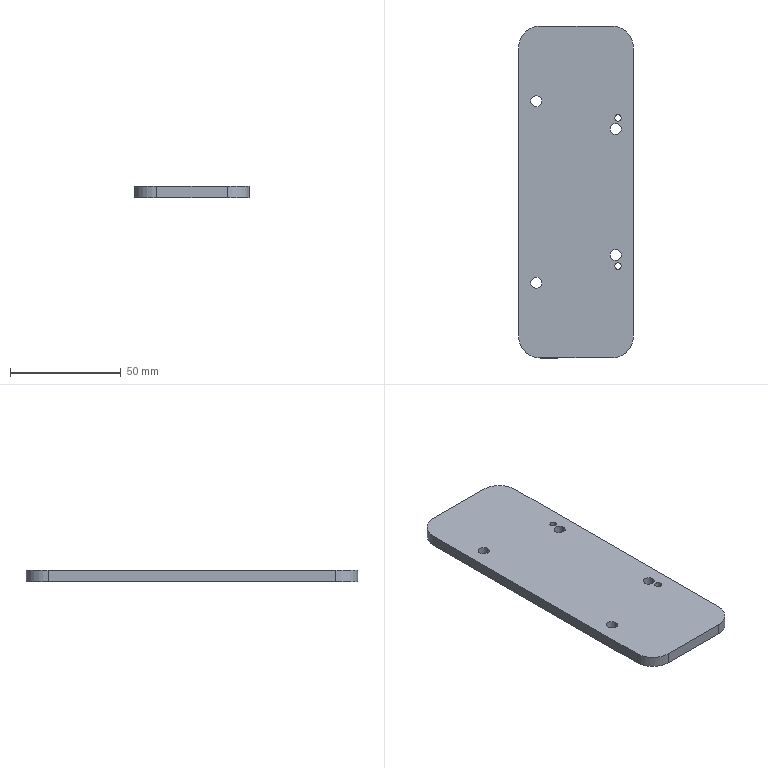Component | SolidWorks | MGL-PACK-03-00Fixture-1_MGL-PACK-03-02MovingPlate-1 | 1 solid | 22 faces | box 52 x 150 x 5 mm | volume 38107 mm3 | cylinder 16 | plane 6 | commonest cylinder face diameters 5 x8 3 x4 20 x4
build123d program:
from build123d import *

# Parameters (mm, degrees)
SKETCH1_W             = 52
SKETCH1_H             = 150
BOSS_EXTRUDE1_DEPTH   = 5
FILLET1_R             = 10
M5_TAPPED_HOLE1_D     = 5
M5_TAPPED_HOLE1_DEPTH = 14
M5_TAPPED_HOLE1_TIP   = 1.502
M3_TAPPED_HOLE1_D     = 3
M3_TAPPED_HOLE1_DEPTH = 8.5
M3_TAPPED_HOLE1_TIP   = 0.9013


with BuildPart() as part:
    # Sketch1 → Boss-Extrude1 (new body)
    with BuildSketch(Plane.XY):
        Rectangle(SKETCH1_W, SKETCH1_H)
    extrude(amount=BOSS_EXTRUDE1_DEPTH)

    # Fillet1
    fillet1_edges = [part.edges().sort_by_distance(p)[0] for p in [
        (-26, 75, 2.5),
        (26, 75, 2.5),
        (26, -75, 2.5),
        (-26, -75, 2.5),
    ]]
    fillet(fillet1_edges, radius=FILLET1_R)

    # M5 Tapped Hole1
    with Locations(Plane(origin=(0, 0, 0), x_dir=(-1, 0, 0), z_dir=(0, 0, -1))):
        with Locations((18, 41), (18, -41), (-18, -28.5), (-18, 28.5)):
            Hole(M5_TAPPED_HOLE1_D / 2, depth=M5_TAPPED_HOLE1_DEPTH)
            with Locations((0, 0, -(M5_TAPPED_HOLE1_DEPTH + M5_TAPPED_HOLE1_TIP / 2))):  # 118° drill point
                Cone(0, M5_TAPPED_HOLE1_D / 2, M5_TAPPED_HOLE1_TIP, mode=Mode.SUBTRACT)

    # M3 Tapped Hole1
    with Locations(Plane(origin=(0, 0, 0), x_dir=(-1, 0, 0), z_dir=(0, 0, -1))):
        with Locations((-19, 33.5), (-19, -33.5)):
            Hole(M3_TAPPED_HOLE1_D / 2, depth=M3_TAPPED_HOLE1_DEPTH)
            with Locations((0, 0, -(M3_TAPPED_HOLE1_DEPTH + M3_TAPPED_HOLE1_TIP / 2))):  # 118° drill point
                Cone(0, M3_TAPPED_HOLE1_D / 2, M3_TAPPED_HOLE1_TIP, mode=Mode.SUBTRACT)


solid = part.part

# Placed as in the assembly
solid = solid.moved(Location((248.5, 0, 13.7), (0, 0, 0)))
STEP:
#1=COLOUR_RGB('',0.7922,0.8196,0.9333);
#2=FILL_AREA_STYLE_COLOUR('',#1);
#3=FILL_AREA_STYLE('',(#2));
#4=SURFACE_STYLE_FILL_AREA(#3);
#5=SURFACE_SIDE_STYLE('',(#4));
#6=SURFACE_STYLE_USAGE(.BOTH.,#5);
#7=PRESENTATION_STYLE_ASSIGNMENT((#6));
#8=CARTESIAN_POINT('',(10.472,-1.319,0.5394));
#9=VERTEX_POINT('',#8);
#10=CARTESIAN_POINT('',(10.591,-1.319,0.5394));
#11=VERTEX_POINT('',#10);
#12=CARTESIAN_POINT('',(10.531,-1.319,0.5394));
#13=DIRECTION('',(-0.,-0.,-1.));
#14=DIRECTION('',(1.,0.,0.));
#15=AXIS2_PLACEMENT_3D('',#12,#13,#14);
#16=CIRCLE('',#15,0.05906);
#17=EDGE_CURVE('',#9,#11,#16,.T.);
#18=ORIENTED_EDGE('',*,*,#17,.T.);
#19=CARTESIAN_POINT('',(10.591,-1.319,0.7362));
#20=VERTEX_POINT('',#19);
#21=CARTESIAN_POINT('',(10.591,-1.319,0.7362));
#22=DIRECTION('',(0.,0.,1.));
#23=VECTOR('',#22,39.37);
#24=LINE('',#21,#23);
#25=EDGE_CURVE('',#11,#20,#24,.T.);
#26=ORIENTED_EDGE('',*,*,#25,.T.);
#27=CARTESIAN_POINT('',(10.472,-1.319,0.7362));
#28=VERTEX_POINT('',#27);
#29=CARTESIAN_POINT('',(10.531,-1.319,0.7362));
#30=DIRECTION('',(0.,0.,1.));
#31=DIRECTION('',(-1.,0.,0.));
#32=AXIS2_PLACEMENT_3D('',#29,#30,#31);
#33=CIRCLE('',#32,0.05906);
#34=EDGE_CURVE('',#20,#28,#33,.T.);
#35=ORIENTED_EDGE('',*,*,#34,.T.);
#36=CARTESIAN_POINT('',(10.472,-1.319,0.7362));
#37=DIRECTION('',(0.,0.,1.));
#38=VECTOR('',#37,39.37);
#39=LINE('',#36,#38);
#40=EDGE_CURVE('',#9,#28,#39,.T.);
#41=ORIENTED_EDGE('',*,*,#40,.F.);
#42=EDGE_LOOP('',(#18,#26,#35,#41));
#43=FACE_OUTER_BOUND('',#42,.T.);
#44=CARTESIAN_POINT('',(10.531,-1.319,0.7362));
#45=DIRECTION('',(0.,0.,1.));
#46=DIRECTION('',(-1.,0.,0.));
#47=AXIS2_PLACEMENT_3D('',#44,#45,#46);
#48=CYLINDRICAL_SURFACE('',#47,0.05906);
#49=ADVANCED_FACE('',(#43),#48,.F.);
#50=CARTESIAN_POINT('',(10.472,1.319,0.5394));
#51=VERTEX_POINT('',#50);
#52=CARTESIAN_POINT('',(10.591,1.319,0.5394));
#53=VERTEX_POINT('',#52);
#54=CARTESIAN_POINT('',(10.531,1.319,0.5394));
#55=DIRECTION('',(-0.,-0.,-1.));
#56=DIRECTION('',(1.,0.,0.));
#57=AXIS2_PLACEMENT_3D('',#54,#55,#56);
#58=CIRCLE('',#57,0.05906);
#59=EDGE_CURVE('',#51,#53,#58,.T.);
#60=ORIENTED_EDGE('',*,*,#59,.T.);
#61=CARTESIAN_POINT('',(10.591,1.319,0.7362));
#62=VERTEX_POINT('',#61);
#63=CARTESIAN_POINT('',(10.591,1.319,0.7362));
#64=DIRECTION('',(0.,0.,1.));
#65=VECTOR('',#64,39.37);
#66=LINE('',#63,#65);
#67=EDGE_CURVE('',#53,#62,#66,.T.);
#68=ORIENTED_EDGE('',*,*,#67,.T.);
#69=CARTESIAN_POINT('',(10.472,1.319,0.7362));
#70=VERTEX_POINT('',#69);
#71=CARTESIAN_POINT('',(10.531,1.319,0.7362));
#72=DIRECTION('',(0.,0.,1.));
#73=DIRECTION('',(-1.,0.,0.));
#74=AXIS2_PLACEMENT_3D('',#71,#72,#73);
#75=CIRCLE('',#74,0.05906);
#76=EDGE_CURVE('',#62,#70,#75,.T.);
#77=ORIENTED_EDGE('',*,*,#76,.T.);
#78=CARTESIAN_POINT('',(10.472,1.319,0.7362));
#79=DIRECTION('',(0.,0.,1.));
#80=VECTOR('',#79,39.37);
#81=LINE('',#78,#80);
#82=EDGE_CURVE('',#51,#70,#81,.T.);
#83=ORIENTED_EDGE('',*,*,#82,.F.);
#84=EDGE_LOOP('',(#60,#68,#77,#83));
#85=FACE_OUTER_BOUND('',#84,.T.);
#86=CARTESIAN_POINT('',(10.531,1.319,0.7362));
#87=DIRECTION('',(0.,0.,1.));
#88=DIRECTION('',(-1.,0.,0.));
#89=AXIS2_PLACEMENT_3D('',#86,#87,#88);
#90=CYLINDRICAL_SURFACE('',#89,0.05906);
#91=ADVANCED_FACE('',(#85),#90,.F.);
#92=CARTESIAN_POINT('',(8.976,-1.614,0.5394));
#93=VERTEX_POINT('',#92);
#94=CARTESIAN_POINT('',(9.173,-1.614,0.5394));
#95=VERTEX_POINT('',#94);
#96=CARTESIAN_POINT('',(9.075,-1.614,0.5394));
#97=DIRECTION('',(-0.,-0.,-1.));
#98=DIRECTION('',(1.,0.,0.));
#99=AXIS2_PLACEMENT_3D('',#96,#97,#98);
#100=CIRCLE('',#99,0.09843);
#101=EDGE_CURVE('',#93,#95,#100,.T.);
#102=ORIENTED_EDGE('',*,*,#101,.T.);
#103=CARTESIAN_POINT('',(9.173,-1.614,0.7362));
#104=VERTEX_POINT('',#103);
#105=CARTESIAN_POINT('',(9.173,-1.614,0.7362));
#106=DIRECTION('',(0.,0.,1.));
#107=VECTOR('',#106,39.37);
#108=LINE('',#105,#107);
#109=EDGE_CURVE('',#95,#104,#108,.T.);
#110=ORIENTED_EDGE('',*,*,#109,.T.);
#111=CARTESIAN_POINT('',(8.976,-1.614,0.7362));
#112=VERTEX_POINT('',#111);
#113=CARTESIAN_POINT('',(9.075,-1.614,0.7362));
#114=DIRECTION('',(0.,0.,1.));
#115=DIRECTION('',(-1.,0.,0.));
#116=AXIS2_PLACEMENT_3D('',#113,#114,#115);
#117=CIRCLE('',#116,0.09843);
#118=EDGE_CURVE('',#104,#112,#117,.T.);
#119=ORIENTED_EDGE('',*,*,#118,.T.);
#120=CARTESIAN_POINT('',(8.976,-1.614,0.7362));
#121=DIRECTION('',(0.,0.,1.));
#122=VECTOR('',#121,39.37);
#123=LINE('',#120,#122);
#124=EDGE_CURVE('',#93,#112,#123,.T.);
#125=ORIENTED_EDGE('',*,*,#124,.F.);
#126=EDGE_LOOP('',(#102,#110,#119,#125));
#127=FACE_OUTER_BOUND('',#126,.T.);
#128=CARTESIAN_POINT('',(9.075,-1.614,0.7362));
#129=DIRECTION('',(0.,0.,1.));
#130=DIRECTION('',(-1.,0.,0.));
#131=AXIS2_PLACEMENT_3D('',#128,#129,#130);
#132=CYLINDRICAL_SURFACE('',#131,0.09843);
#133=ADVANCED_FACE('',(#127),#132,.F.);
#134=CARTESIAN_POINT('',(8.976,1.614,0.5394));
#135=VERTEX_POINT('',#134);
#136=CARTESIAN_POINT('',(9.173,1.614,0.5394));
#137=VERTEX_POINT('',#136);
#138=CARTESIAN_POINT('',(9.075,1.614,0.5394));
#139=DIRECTION('',(-0.,-0.,-1.));
#140=DIRECTION('',(1.,0.,0.));
#141=AXIS2_PLACEMENT_3D('',#138,#139,#140);
#142=CIRCLE('',#141,0.09843);
#143=EDGE_CURVE('',#135,#137,#142,.T.);
#144=ORIENTED_EDGE('',*,*,#143,.T.);
#145=CARTESIAN_POINT('',(9.173,1.614,0.7362));
#146=VERTEX_POINT('',#145);
#147=CARTESIAN_POINT('',(9.173,1.614,0.7362));
#148=DIRECTION('',(0.,0.,1.));
#149=VECTOR('',#148,39.37);
#150=LINE('',#147,#149);
#151=EDGE_CURVE('',#137,#146,#150,.T.);
#152=ORIENTED_EDGE('',*,*,#151,.T.);
#153=CARTESIAN_POINT('',(8.976,1.614,0.7362));
#154=VERTEX_POINT('',#153);
#155=CARTESIAN_POINT('',(9.075,1.614,0.7362));
#156=DIRECTION('',(0.,0.,1.));
#157=DIRECTION('',(-1.,0.,0.));
#158=AXIS2_PLACEMENT_3D('',#155,#156,#157);
#159=CIRCLE('',#158,0.09843);
#160=EDGE_CURVE('',#146,#154,#159,.T.);
#161=ORIENTED_EDGE('',*,*,#160,.T.);
#162=CARTESIAN_POINT('',(8.976,1.614,0.7362));
#163=DIRECTION('',(0.,0.,1.));
#164=VECTOR('',#163,39.37);
#165=LINE('',#162,#164);
#166=EDGE_CURVE('',#135,#154,#165,.T.);
#167=ORIENTED_EDGE('',*,*,#166,.F.);
#168=EDGE_LOOP('',(#144,#152,#161,#167));
#169=FACE_OUTER_BOUND('',#168,.T.);
#170=CARTESIAN_POINT('',(9.075,1.614,0.7362));
#171=DIRECTION('',(0.,0.,1.));
#172=DIRECTION('',(-1.,0.,0.));
#173=AXIS2_PLACEMENT_3D('',#170,#171,#172);
#174=CYLINDRICAL_SURFACE('',#173,0.09843);
#175=ADVANCED_FACE('',(#169),#174,.F.);
#176=CARTESIAN_POINT('',(10.394,1.122,0.5394));
#177=VERTEX_POINT('',#176);
#178=CARTESIAN_POINT('',(10.591,1.122,0.5394));
#179=VERTEX_POINT('',#178);
#180=CARTESIAN_POINT('',(10.492,1.122,0.5394));
#181=DIRECTION('',(-0.,-0.,-1.));
#182=DIRECTION('',(1.,0.,0.));
#183=AXIS2_PLACEMENT_3D('',#180,#181,#182);
#184=CIRCLE('',#183,0.09843);
#185=EDGE_CURVE('',#177,#179,#184,.T.);
#186=ORIENTED_EDGE('',*,*,#185,.T.);
#187=CARTESIAN_POINT('',(10.591,1.122,0.7362));
#188=VERTEX_POINT('',#187);
#189=CARTESIAN_POINT('',(10.591,1.122,0.7362));
#190=DIRECTION('',(0.,0.,1.));
#191=VECTOR('',#190,39.37);
#192=LINE('',#189,#191);
#193=EDGE_CURVE('',#179,#188,#192,.T.);
#194=ORIENTED_EDGE('',*,*,#193,.T.);
#195=CARTESIAN_POINT('',(10.394,1.122,0.7362));
#196=VERTEX_POINT('',#195);
#197=CARTESIAN_POINT('',(10.492,1.122,0.7362));
#198=DIRECTION('',(0.,0.,1.));
#199=DIRECTION('',(-1.,0.,0.));
#200=AXIS2_PLACEMENT_3D('',#197,#198,#199);
#201=CIRCLE('',#200,0.09843);
#202=EDGE_CURVE('',#188,#196,#201,.T.);
#203=ORIENTED_EDGE('',*,*,#202,.T.);
#204=CARTESIAN_POINT('',(10.394,1.122,0.7362));
#205=DIRECTION('',(0.,0.,1.));
#206=VECTOR('',#205,39.37);
#207=LINE('',#204,#206);
#208=EDGE_CURVE('',#177,#196,#207,.T.);
#209=ORIENTED_EDGE('',*,*,#208,.F.);
#210=EDGE_LOOP('',(#186,#194,#203,#209));
#211=FACE_OUTER_BOUND('',#210,.T.);
#212=CARTESIAN_POINT('',(10.492,1.122,0.7362));
#213=DIRECTION('',(0.,0.,1.));
#214=DIRECTION('',(-1.,0.,0.));
#215=AXIS2_PLACEMENT_3D('',#212,#213,#214);
#216=CYLINDRICAL_SURFACE('',#215,0.09843);
#217=ADVANCED_FACE('',(#211),#216,.F.);
#218=CARTESIAN_POINT('',(10.394,-1.122,0.5394));
#219=VERTEX_POINT('',#218);
#220=CARTESIAN_POINT('',(10.591,-1.122,0.5394));
#221=VERTEX_POINT('',#220);
#222=CARTESIAN_POINT('',(10.492,-1.122,0.5394));
#223=DIRECTION('',(-0.,-0.,-1.));
#224=DIRECTION('',(1.,0.,0.));
#225=AXIS2_PLACEMENT_3D('',#222,#223,#224);
#226=CIRCLE('',#225,0.09843);
#227=EDGE_CURVE('',#219,#221,#226,.T.);
#228=ORIENTED_EDGE('',*,*,#227,.T.);
#229=CARTESIAN_POINT('',(10.591,-1.122,0.7362));
#230=VERTEX_POINT('',#229);
#231=CARTESIAN_POINT('',(10.591,-1.122,0.7362));
#232=DIRECTION('',(0.,0.,1.));
#233=VECTOR('',#232,39.37);
#234=LINE('',#231,#233);
#235=EDGE_CURVE('',#221,#230,#234,.T.);
#236=ORIENTED_EDGE('',*,*,#235,.T.);
#237=CARTESIAN_POINT('',(10.394,-1.122,0.7362));
#238=VERTEX_POINT('',#237);
#239=CARTESIAN_POINT('',(10.492,-1.122,0.7362));
#240=DIRECTION('',(0.,0.,1.));
#241=DIRECTION('',(-1.,0.,0.));
#242=AXIS2_PLACEMENT_3D('',#239,#240,#241);
#243=CIRCLE('',#242,0.09843);
#244=EDGE_CURVE('',#230,#238,#243,.T.);
#245=ORIENTED_EDGE('',*,*,#244,.T.);
#246=CARTESIAN_POINT('',(10.394,-1.122,0.7362));
#247=DIRECTION('',(0.,0.,1.));
#248=VECTOR('',#247,39.37);
#249=LINE('',#246,#248);
#250=EDGE_CURVE('',#219,#238,#249,.T.);
#251=ORIENTED_EDGE('',*,*,#250,.F.);
#252=EDGE_LOOP('',(#228,#236,#245,#251));
#253=FACE_OUTER_BOUND('',#252,.T.);
#254=CARTESIAN_POINT('',(10.492,-1.122,0.7362));
#255=DIRECTION('',(0.,0.,1.));
#256=DIRECTION('',(-1.,0.,0.));
#257=AXIS2_PLACEMENT_3D('',#254,#255,#256);
#258=CYLINDRICAL_SURFACE('',#257,0.09843);
#259=ADVANCED_FACE('',(#253),#258,.F.);
#260=CARTESIAN_POINT('',(8.76,-2.559,0.7362));
#261=VERTEX_POINT('',#260);
#262=CARTESIAN_POINT('',(8.76,2.559,0.7362));
#263=VERTEX_POINT('',#262);
#264=CARTESIAN_POINT('',(8.76,-2.953,0.7362));
#265=DIRECTION('',(-0.,1.,-0.));
#266=VECTOR('',#265,39.37);
#267=LINE('',#264,#266);
#268=EDGE_CURVE('',#261,#263,#267,.T.);
#269=ORIENTED_EDGE('',*,*,#268,.T.);
#270=CARTESIAN_POINT('',(8.76,2.559,0.5394));
#271=VERTEX_POINT('',#270);
#272=CARTESIAN_POINT('',(8.76,2.559,0.5394));
#273=DIRECTION('',(-0.,-0.,-1.));
#274=VECTOR('',#273,39.37);
#275=LINE('',#272,#274);
#276=EDGE_CURVE('',#263,#271,#275,.T.);
#277=ORIENTED_EDGE('',*,*,#276,.T.);
#278=CARTESIAN_POINT('',(8.76,-2.559,0.5394));
#279=VERTEX_POINT('',#278);
#280=CARTESIAN_POINT('',(8.76,-2.953,0.5394));
#281=DIRECTION('',(-0.,1.,-0.));
#282=VECTOR('',#281,39.37);
#283=LINE('',#280,#282);
#284=EDGE_CURVE('',#279,#271,#283,.T.);
#285=ORIENTED_EDGE('',*,*,#284,.F.);
#286=CARTESIAN_POINT('',(8.76,-2.559,0.5394));
#287=DIRECTION('',(0.,0.,1.));
#288=VECTOR('',#287,39.37);
#289=LINE('',#286,#288);
#290=EDGE_CURVE('',#279,#261,#289,.T.);
#291=ORIENTED_EDGE('',*,*,#290,.T.);
#292=EDGE_LOOP('',(#269,#277,#285,#291));
#293=FACE_OUTER_BOUND('',#292,.T.);
#294=CARTESIAN_POINT('',(8.76,-2.953,0.5394));
#295=DIRECTION('',(1.,0.,-0.));
#296=DIRECTION('',(0.,-1.,0.));
#297=AXIS2_PLACEMENT_3D('',#294,#295,#296);
#298=PLANE('',#297);
#299=ADVANCED_FACE('',(#293),#298,.F.);
#300=CARTESIAN_POINT('',(9.154,2.953,0.7362));
#301=VERTEX_POINT('',#300);
#302=CARTESIAN_POINT('',(10.413,2.953,0.7362));
#303=VERTEX_POINT('',#302);
#304=CARTESIAN_POINT('',(8.76,2.953,0.7362));
#305=DIRECTION('',(1.,0.,-0.));
#306=VECTOR('',#305,39.37);
#307=LINE('',#304,#306);
#308=EDGE_CURVE('',#301,#303,#307,.T.);
#309=ORIENTED_EDGE('',*,*,#308,.T.);
#310=CARTESIAN_POINT('',(10.413,2.953,0.5394));
#311=VERTEX_POINT('',#310);
#312=CARTESIAN_POINT('',(10.413,2.953,0.5394));
#313=DIRECTION('',(-0.,-0.,-1.));
#314=VECTOR('',#313,39.37);
#315=LINE('',#312,#314);
#316=EDGE_CURVE('',#303,#311,#315,.T.);
#317=ORIENTED_EDGE('',*,*,#316,.T.);
#318=CARTESIAN_POINT('',(9.154,2.953,0.5394));
#319=VERTEX_POINT('',#318);
#320=CARTESIAN_POINT('',(8.76,2.953,0.5394));
#321=DIRECTION('',(1.,0.,-0.));
#322=VECTOR('',#321,39.37);
#323=LINE('',#320,#322);
#324=EDGE_CURVE('',#319,#311,#323,.T.);
#325=ORIENTED_EDGE('',*,*,#324,.F.);
#326=CARTESIAN_POINT('',(9.154,2.953,0.5394));
#327=DIRECTION('',(0.,0.,1.));
#328=VECTOR('',#327,39.37);
#329=LINE('',#326,#328);
#330=EDGE_CURVE('',#319,#301,#329,.T.);
#331=ORIENTED_EDGE('',*,*,#330,.T.);
#332=EDGE_LOOP('',(#309,#317,#325,#331));
#333=FACE_OUTER_BOUND('',#332,.T.);
#334=CARTESIAN_POINT('',(8.76,2.953,0.5394));
#335=DIRECTION('',(0.,-1.,0.));
#336=DIRECTION('',(-0.,-0.,-1.));
#337=AXIS2_PLACEMENT_3D('',#334,#335,#336);
#338=PLANE('',#337);
#339=ADVANCED_FACE('',(#333),#338,.F.);
#340=CARTESIAN_POINT('',(10.807,2.559,0.5394));
#341=VERTEX_POINT('',#340);
#342=CARTESIAN_POINT('',(10.807,-2.559,0.5394));
#343=VERTEX_POINT('',#342);
#344=CARTESIAN_POINT('',(10.807,-2.953,0.5394));
#345=DIRECTION('',(0.,-1.,0.));
#346=VECTOR('',#345,39.37);
#347=LINE('',#344,#346);
#348=EDGE_CURVE('',#341,#343,#347,.T.);
#349=ORIENTED_EDGE('',*,*,#348,.F.);
#350=CARTESIAN_POINT('',(10.807,2.559,0.7362));
#351=VERTEX_POINT('',#350);
#352=CARTESIAN_POINT('',(10.807,2.559,0.5394));
#353=DIRECTION('',(0.,0.,1.));
#354=VECTOR('',#353,39.37);
#355=LINE('',#352,#354);
#356=EDGE_CURVE('',#341,#351,#355,.T.);
#357=ORIENTED_EDGE('',*,*,#356,.T.);
#358=CARTESIAN_POINT('',(10.807,-2.559,0.7362));
#359=VERTEX_POINT('',#358);
#360=CARTESIAN_POINT('',(10.807,-2.953,0.7362));
#361=DIRECTION('',(0.,-1.,0.));
#362=VECTOR('',#361,39.37);
#363=LINE('',#360,#362);
#364=EDGE_CURVE('',#351,#359,#363,.T.);
#365=ORIENTED_EDGE('',*,*,#364,.T.);
#366=CARTESIAN_POINT('',(10.807,-2.559,0.5394));
#367=DIRECTION('',(-0.,-0.,-1.));
#368=VECTOR('',#367,39.37);
#369=LINE('',#366,#368);
#370=EDGE_CURVE('',#359,#343,#369,.T.);
#371=ORIENTED_EDGE('',*,*,#370,.T.);
#372=EDGE_LOOP('',(#349,#357,#365,#371));
#373=FACE_OUTER_BOUND('',#372,.T.);
#374=CARTESIAN_POINT('',(10.807,-2.953,0.5394));
#375=DIRECTION('',(-1.,-0.,0.));
#376=DIRECTION('',(-0.,1.,-0.));
#377=AXIS2_PLACEMENT_3D('',#374,#375,#376);
#378=PLANE('',#377);
#379=ADVANCED_FACE('',(#373),#378,.F.);
#380=CARTESIAN_POINT('',(10.413,-2.953,0.7362));
#381=VERTEX_POINT('',#380);
#382=CARTESIAN_POINT('',(9.154,-2.953,0.7362));
#383=VERTEX_POINT('',#382);
#384=CARTESIAN_POINT('',(8.76,-2.953,0.7362));
#385=DIRECTION('',(-1.,-0.,0.));
#386=VECTOR('',#385,39.37);
#387=LINE('',#384,#386);
#388=EDGE_CURVE('',#381,#383,#387,.T.);
#389=ORIENTED_EDGE('',*,*,#388,.T.);
#390=CARTESIAN_POINT('',(9.154,-2.953,0.5394));
#391=VERTEX_POINT('',#390);
#392=CARTESIAN_POINT('',(9.154,-2.953,0.5394));
#393=DIRECTION('',(-0.,-0.,-1.));
#394=VECTOR('',#393,39.37);
#395=LINE('',#392,#394);
#396=EDGE_CURVE('',#383,#391,#395,.T.);
#397=ORIENTED_EDGE('',*,*,#396,.T.);
#398=CARTESIAN_POINT('',(10.413,-2.953,0.5394));
#399=VERTEX_POINT('',#398);
#400=CARTESIAN_POINT('',(8.76,-2.953,0.5394));
#401=DIRECTION('',(-1.,-0.,0.));
#402=VECTOR('',#401,39.37);
#403=LINE('',#400,#402);
#404=EDGE_CURVE('',#399,#391,#403,.T.);
#405=ORIENTED_EDGE('',*,*,#404,.F.);
#406=CARTESIAN_POINT('',(10.413,-2.953,0.5394));
#407=DIRECTION('',(0.,0.,1.));
#408=VECTOR('',#407,39.37);
#409=LINE('',#406,#408);
#410=EDGE_CURVE('',#399,#381,#409,.T.);
#411=ORIENTED_EDGE('',*,*,#410,.T.);
#412=EDGE_LOOP('',(#389,#397,#405,#411));
#413=FACE_OUTER_BOUND('',#412,.T.);
#414=CARTESIAN_POINT('',(8.76,-2.953,0.5394));
#415=DIRECTION('',(-0.,1.,-0.));
#416=DIRECTION('',(0.,0.,1.));
#417=AXIS2_PLACEMENT_3D('',#414,#415,#416);
#418=PLANE('',#417);
#419=ADVANCED_FACE('',(#413),#418,.F.);
#420=ORIENTED_EDGE('',*,*,#17,.F.);
#421=CARTESIAN_POINT('',(10.531,-1.319,0.5394));
#422=DIRECTION('',(-0.,-0.,-1.));
#423=DIRECTION('',(1.,0.,0.));
#424=AXIS2_PLACEMENT_3D('',#421,#422,#423);
#425=CIRCLE('',#424,0.05906);
#426=EDGE_CURVE('',#11,#9,#425,.T.);
#427=ORIENTED_EDGE('',*,*,#426,.F.);
#428=EDGE_LOOP('',(#420,#427));
#429=FACE_BOUND('',#428,.T.);
#430=ORIENTED_EDGE('',*,*,#59,.F.);
#431=CARTESIAN_POINT('',(10.531,1.319,0.5394));
#432=DIRECTION('',(-0.,-0.,-1.));
#433=DIRECTION('',(1.,0.,0.));
#434=AXIS2_PLACEMENT_3D('',#431,#432,#433);
#435=CIRCLE('',#434,0.05906);
#436=EDGE_CURVE('',#53,#51,#435,.T.);
#437=ORIENTED_EDGE('',*,*,#436,.F.);
#438=EDGE_LOOP('',(#430,#437));
#439=FACE_BOUND('',#438,.T.);
#440=ORIENTED_EDGE('',*,*,#101,.F.);
#441=CARTESIAN_POINT('',(9.075,-1.614,0.5394));
#442=DIRECTION('',(-0.,-0.,-1.));
#443=DIRECTION('',(1.,0.,0.));
#444=AXIS2_PLACEMENT_3D('',#441,#442,#443);
#445=CIRCLE('',#444,0.09843);
#446=EDGE_CURVE('',#95,#93,#445,.T.);
#447=ORIENTED_EDGE('',*,*,#446,.F.);
#448=EDGE_LOOP('',(#440,#447));
#449=FACE_BOUND('',#448,.T.);
#450=ORIENTED_EDGE('',*,*,#143,.F.);
#451=CARTESIAN_POINT('',(9.075,1.614,0.5394));
#452=DIRECTION('',(-0.,-0.,-1.));
#453=DIRECTION('',(1.,0.,0.));
#454=AXIS2_PLACEMENT_3D('',#451,#452,#453);
#455=CIRCLE('',#454,0.09843);
#456=EDGE_CURVE('',#137,#135,#455,.T.);
#457=ORIENTED_EDGE('',*,*,#456,.F.);
#458=EDGE_LOOP('',(#450,#457));
#459=FACE_BOUND('',#458,.T.);
#460=ORIENTED_EDGE('',*,*,#185,.F.);
#461=CARTESIAN_POINT('',(10.492,1.122,0.5394));
#462=DIRECTION('',(-0.,-0.,-1.));
#463=DIRECTION('',(1.,0.,0.));
#464=AXIS2_PLACEMENT_3D('',#461,#462,#463);
#465=CIRCLE('',#464,0.09843);
#466=EDGE_CURVE('',#179,#177,#465,.T.);
#467=ORIENTED_EDGE('',*,*,#466,.F.);
#468=EDGE_LOOP('',(#460,#467));
#469=FACE_BOUND('',#468,.T.);
#470=ORIENTED_EDGE('',*,*,#227,.F.);
#471=CARTESIAN_POINT('',(10.492,-1.122,0.5394));
#472=DIRECTION('',(-0.,-0.,-1.));
#473=DIRECTION('',(1.,0.,0.));
#474=AXIS2_PLACEMENT_3D('',#471,#472,#473);
#475=CIRCLE('',#474,0.09843);
#476=EDGE_CURVE('',#221,#219,#475,.T.);
#477=ORIENTED_EDGE('',*,*,#476,.F.);
#478=EDGE_LOOP('',(#470,#477));
#479=FACE_BOUND('',#478,.T.);
#480=ORIENTED_EDGE('',*,*,#324,.T.);
#481=CARTESIAN_POINT('',(10.413,2.559,0.5394));
#482=DIRECTION('',(-0.,-0.,-1.));
#483=DIRECTION('',(1.,0.,0.));
#484=AXIS2_PLACEMENT_3D('',#481,#482,#483);
#485=CIRCLE('',#484,0.3937);
#486=EDGE_CURVE('',#311,#341,#485,.T.);
#487=ORIENTED_EDGE('',*,*,#486,.T.);
#488=ORIENTED_EDGE('',*,*,#348,.T.);
#489=CARTESIAN_POINT('',(10.413,-2.559,0.5394));
#490=DIRECTION('',(-0.,-0.,-1.));
#491=DIRECTION('',(1.,0.,0.));
#492=AXIS2_PLACEMENT_3D('',#489,#490,#491);
#493=CIRCLE('',#492,0.3937);
#494=EDGE_CURVE('',#343,#399,#493,.T.);
#495=ORIENTED_EDGE('',*,*,#494,.T.);
#496=ORIENTED_EDGE('',*,*,#404,.T.);
#497=CARTESIAN_POINT('',(9.154,-2.559,0.5394));
#498=DIRECTION('',(-0.,-0.,-1.));
#499=DIRECTION('',(1.,0.,0.));
#500=AXIS2_PLACEMENT_3D('',#497,#498,#499);
#501=CIRCLE('',#500,0.3937);
#502=EDGE_CURVE('',#391,#279,#501,.T.);
#503=ORIENTED_EDGE('',*,*,#502,.T.);
#504=ORIENTED_EDGE('',*,*,#284,.T.);
#505=CARTESIAN_POINT('',(9.154,2.559,0.5394));
#506=DIRECTION('',(-0.,-0.,-1.));
#507=DIRECTION('',(1.,0.,0.));
#508=AXIS2_PLACEMENT_3D('',#505,#506,#507);
#509=CIRCLE('',#508,0.3937);
#510=EDGE_CURVE('',#271,#319,#509,.T.);
#511=ORIENTED_EDGE('',*,*,#510,.T.);
#512=EDGE_LOOP('',(#480,#487,#488,#495,#496,#503,#504,#511));
#513=FACE_OUTER_BOUND('',#512,.T.);
#514=CARTESIAN_POINT('',(9.783,0.,0.5394));
#515=DIRECTION('',(-0.,-0.,-1.));
#516=DIRECTION('',(1.,0.,-0.));
#517=AXIS2_PLACEMENT_3D('',#514,#515,#516);
#518=PLANE('',#517);
#519=ADVANCED_FACE('',(#429,#439,#449,#459,#469,#479,#513),#518,.T.);
#520=CARTESIAN_POINT('',(10.531,-1.319,0.7362));
#521=DIRECTION('',(0.,0.,1.));
#522=DIRECTION('',(-1.,0.,0.));
#523=AXIS2_PLACEMENT_3D('',#520,#521,#522);
#524=CIRCLE('',#523,0.05906);
#525=EDGE_CURVE('',#28,#20,#524,.T.);
#526=ORIENTED_EDGE('',*,*,#525,.F.);
#527=ORIENTED_EDGE('',*,*,#34,.F.);
#528=EDGE_LOOP('',(#526,#527));
#529=FACE_BOUND('',#528,.T.);
#530=CARTESIAN_POINT('',(10.531,1.319,0.7362));
#531=DIRECTION('',(0.,0.,1.));
#532=DIRECTION('',(-1.,0.,0.));
#533=AXIS2_PLACEMENT_3D('',#530,#531,#532);
#534=CIRCLE('',#533,0.05906);
#535=EDGE_CURVE('',#70,#62,#534,.T.);
#536=ORIENTED_EDGE('',*,*,#535,.F.);
#537=ORIENTED_EDGE('',*,*,#76,.F.);
#538=EDGE_LOOP('',(#536,#537));
#539=FACE_BOUND('',#538,.T.);
#540=CARTESIAN_POINT('',(9.075,-1.614,0.7362));
#541=DIRECTION('',(0.,0.,1.));
#542=DIRECTION('',(-1.,0.,0.));
#543=AXIS2_PLACEMENT_3D('',#540,#541,#542);
#544=CIRCLE('',#543,0.09843);
#545=EDGE_CURVE('',#112,#104,#544,.T.);
#546=ORIENTED_EDGE('',*,*,#545,.F.);
#547=ORIENTED_EDGE('',*,*,#118,.F.);
#548=EDGE_LOOP('',(#546,#547));
#549=FACE_BOUND('',#548,.T.);
#550=CARTESIAN_POINT('',(9.075,1.614,0.7362));
#551=DIRECTION('',(0.,0.,1.));
#552=DIRECTION('',(-1.,0.,0.));
#553=AXIS2_PLACEMENT_3D('',#550,#551,#552);
#554=CIRCLE('',#553,0.09843);
#555=EDGE_CURVE('',#154,#146,#554,.T.);
#556=ORIENTED_EDGE('',*,*,#555,.F.);
#557=ORIENTED_EDGE('',*,*,#160,.F.);
#558=EDGE_LOOP('',(#556,#557));
#559=FACE_BOUND('',#558,.T.);
#560=CARTESIAN_POINT('',(10.492,1.122,0.7362));
#561=DIRECTION('',(0.,0.,1.));
#562=DIRECTION('',(-1.,0.,0.));
#563=AXIS2_PLACEMENT_3D('',#560,#561,#562);
#564=CIRCLE('',#563,0.09843);
#565=EDGE_CURVE('',#196,#188,#564,.T.);
#566=ORIENTED_EDGE('',*,*,#565,.F.);
#567=ORIENTED_EDGE('',*,*,#202,.F.);
#568=EDGE_LOOP('',(#566,#567));
#569=FACE_BOUND('',#568,.T.);
#570=CARTESIAN_POINT('',(10.492,-1.122,0.7362));
#571=DIRECTION('',(0.,0.,1.));
#572=DIRECTION('',(-1.,0.,0.));
#573=AXIS2_PLACEMENT_3D('',#570,#571,#572);
#574=CIRCLE('',#573,0.09843);
#575=EDGE_CURVE('',#238,#230,#574,.T.);
#576=ORIENTED_EDGE('',*,*,#575,.F.);
#577=ORIENTED_EDGE('',*,*,#244,.F.);
#578=EDGE_LOOP('',(#576,#577));
#579=FACE_BOUND('',#578,.T.);
#580=ORIENTED_EDGE('',*,*,#364,.F.);
#581=CARTESIAN_POINT('',(10.413,2.559,0.7362));
#582=DIRECTION('',(0.,0.,1.));
#583=DIRECTION('',(1.,0.,0.));
#584=AXIS2_PLACEMENT_3D('',#581,#582,#583);
#585=CIRCLE('',#584,0.3937);
#586=EDGE_CURVE('',#351,#303,#585,.T.);
#587=ORIENTED_EDGE('',*,*,#586,.T.);
#588=ORIENTED_EDGE('',*,*,#308,.F.);
#589=CARTESIAN_POINT('',(9.154,2.559,0.7362));
#590=DIRECTION('',(0.,0.,1.));
#591=DIRECTION('',(1.,0.,0.));
#592=AXIS2_PLACEMENT_3D('',#589,#590,#591);
#593=CIRCLE('',#592,0.3937);
#594=EDGE_CURVE('',#301,#263,#593,.T.);
#595=ORIENTED_EDGE('',*,*,#594,.T.);
#596=ORIENTED_EDGE('',*,*,#268,.F.);
#597=CARTESIAN_POINT('',(9.154,-2.559,0.7362));
#598=DIRECTION('',(0.,0.,1.));
#599=DIRECTION('',(1.,0.,0.));
#600=AXIS2_PLACEMENT_3D('',#597,#598,#599);
#601=CIRCLE('',#600,0.3937);
#602=EDGE_CURVE('',#261,#383,#601,.T.);
#603=ORIENTED_EDGE('',*,*,#602,.T.);
#604=ORIENTED_EDGE('',*,*,#388,.F.);
#605=CARTESIAN_POINT('',(10.413,-2.559,0.7362));
#606=DIRECTION('',(0.,0.,1.));
#607=DIRECTION('',(1.,0.,0.));
#608=AXIS2_PLACEMENT_3D('',#605,#606,#607);
#609=CIRCLE('',#608,0.3937);
#610=EDGE_CURVE('',#381,#359,#609,.T.);
#611=ORIENTED_EDGE('',*,*,#610,.T.);
#612=EDGE_LOOP('',(#580,#587,#588,#595,#596,#603,#604,#611));
#613=FACE_OUTER_BOUND('',#612,.T.);
#614=CARTESIAN_POINT('',(9.783,0.,0.7362));
#615=DIRECTION('',(-0.,-0.,-1.));
#616=DIRECTION('',(1.,0.,-0.));
#617=AXIS2_PLACEMENT_3D('',#614,#615,#616);
#618=PLANE('',#617);
#619=ADVANCED_FACE('',(#529,#539,#549,#559,#569,#579,#613),#618,.F.);
#620=ORIENTED_EDGE('',*,*,#486,.F.);
#621=ORIENTED_EDGE('',*,*,#316,.F.);
#622=ORIENTED_EDGE('',*,*,#586,.F.);
#623=ORIENTED_EDGE('',*,*,#356,.F.);
#624=EDGE_LOOP('',(#620,#621,#622,#623));
#625=FACE_OUTER_BOUND('',#624,.T.);
#626=CARTESIAN_POINT('',(10.413,2.559,0.5394));
#627=DIRECTION('',(0.,0.,1.));
#628=DIRECTION('',(-1.,0.,0.));
#629=AXIS2_PLACEMENT_3D('',#626,#627,#628);
#630=CYLINDRICAL_SURFACE('',#629,0.3937);
#631=ADVANCED_FACE('',(#625),#630,.T.);
#632=ORIENTED_EDGE('',*,*,#510,.F.);
#633=ORIENTED_EDGE('',*,*,#276,.F.);
#634=ORIENTED_EDGE('',*,*,#594,.F.);
#635=ORIENTED_EDGE('',*,*,#330,.F.);
#636=EDGE_LOOP('',(#632,#633,#634,#635));
#637=FACE_OUTER_BOUND('',#636,.T.);
#638=CARTESIAN_POINT('',(9.154,2.559,0.5394));
#639=DIRECTION('',(0.,0.,1.));
#640=DIRECTION('',(-1.,0.,0.));
#641=AXIS2_PLACEMENT_3D('',#638,#639,#640);
#642=CYLINDRICAL_SURFACE('',#641,0.3937);
#643=ADVANCED_FACE('',(#637),#642,.T.);
#644=ORIENTED_EDGE('',*,*,#502,.F.);
#645=ORIENTED_EDGE('',*,*,#396,.F.);
#646=ORIENTED_EDGE('',*,*,#602,.F.);
#647=ORIENTED_EDGE('',*,*,#290,.F.);
#648=EDGE_LOOP('',(#644,#645,#646,#647));
#649=FACE_OUTER_BOUND('',#648,.T.);
#650=CARTESIAN_POINT('',(9.154,-2.559,0.5394));
#651=DIRECTION('',(0.,0.,1.));
#652=DIRECTION('',(-1.,0.,0.));
#653=AXIS2_PLACEMENT_3D('',#650,#651,#652);
#654=CYLINDRICAL_SURFACE('',#653,0.3937);
#655=ADVANCED_FACE('',(#649),#654,.T.);
#656=ORIENTED_EDGE('',*,*,#494,.F.);
#657=ORIENTED_EDGE('',*,*,#370,.F.);
#658=ORIENTED_EDGE('',*,*,#610,.F.);
#659=ORIENTED_EDGE('',*,*,#410,.F.);
#660=EDGE_LOOP('',(#656,#657,#658,#659));
#661=FACE_OUTER_BOUND('',#660,.T.);
#662=CARTESIAN_POINT('',(10.413,-2.559,0.5394));
#663=DIRECTION('',(0.,0.,1.));
#664=DIRECTION('',(-1.,0.,0.));
#665=AXIS2_PLACEMENT_3D('',#662,#663,#664);
#666=CYLINDRICAL_SURFACE('',#665,0.3937);
#667=ADVANCED_FACE('',(#661),#666,.T.);
#668=ORIENTED_EDGE('',*,*,#235,.F.);
#669=ORIENTED_EDGE('',*,*,#476,.T.);
#670=ORIENTED_EDGE('',*,*,#250,.T.);
#671=ORIENTED_EDGE('',*,*,#575,.T.);
#672=EDGE_LOOP('',(#668,#669,#670,#671));
#673=FACE_OUTER_BOUND('',#672,.T.);
#674=CARTESIAN_POINT('',(10.492,-1.122,0.7362));
#675=DIRECTION('',(0.,0.,1.));
#676=DIRECTION('',(-1.,0.,0.));
#677=AXIS2_PLACEMENT_3D('',#674,#675,#676);
#678=CYLINDRICAL_SURFACE('',#677,0.09843);
#679=ADVANCED_FACE('',(#673),#678,.F.);
#680=ORIENTED_EDGE('',*,*,#193,.F.);
#681=ORIENTED_EDGE('',*,*,#466,.T.);
#682=ORIENTED_EDGE('',*,*,#208,.T.);
#683=ORIENTED_EDGE('',*,*,#565,.T.);
#684=EDGE_LOOP('',(#680,#681,#682,#683));
#685=FACE_OUTER_BOUND('',#684,.T.);
#686=CARTESIAN_POINT('',(10.492,1.122,0.7362));
#687=DIRECTION('',(0.,0.,1.));
#688=DIRECTION('',(-1.,0.,0.));
#689=AXIS2_PLACEMENT_3D('',#686,#687,#688);
#690=CYLINDRICAL_SURFACE('',#689,0.09843);
#691=ADVANCED_FACE('',(#685),#690,.F.);
#692=ORIENTED_EDGE('',*,*,#151,.F.);
#693=ORIENTED_EDGE('',*,*,#456,.T.);
#694=ORIENTED_EDGE('',*,*,#166,.T.);
#695=ORIENTED_EDGE('',*,*,#555,.T.);
#696=EDGE_LOOP('',(#692,#693,#694,#695));
#697=FACE_OUTER_BOUND('',#696,.T.);
#698=CARTESIAN_POINT('',(9.075,1.614,0.7362));
#699=DIRECTION('',(0.,0.,1.));
#700=DIRECTION('',(-1.,0.,0.));
#701=AXIS2_PLACEMENT_3D('',#698,#699,#700);
#702=CYLINDRICAL_SURFACE('',#701,0.09843);
#703=ADVANCED_FACE('',(#697),#702,.F.);
#704=ORIENTED_EDGE('',*,*,#109,.F.);
#705=ORIENTED_EDGE('',*,*,#446,.T.);
#706=ORIENTED_EDGE('',*,*,#124,.T.);
#707=ORIENTED_EDGE('',*,*,#545,.T.);
#708=EDGE_LOOP('',(#704,#705,#706,#707));
#709=FACE_OUTER_BOUND('',#708,.T.);
#710=CARTESIAN_POINT('',(9.075,-1.614,0.7362));
#711=DIRECTION('',(0.,0.,1.));
#712=DIRECTION('',(-1.,0.,0.));
#713=AXIS2_PLACEMENT_3D('',#710,#711,#712);
#714=CYLINDRICAL_SURFACE('',#713,0.09843);
#715=ADVANCED_FACE('',(#709),#714,.F.);
#716=ORIENTED_EDGE('',*,*,#67,.F.);
#717=ORIENTED_EDGE('',*,*,#436,.T.);
#718=ORIENTED_EDGE('',*,*,#82,.T.);
#719=ORIENTED_EDGE('',*,*,#535,.T.);
#720=EDGE_LOOP('',(#716,#717,#718,#719));
#721=FACE_OUTER_BOUND('',#720,.T.);
#722=CARTESIAN_POINT('',(10.531,1.319,0.7362));
#723=DIRECTION('',(0.,0.,1.));
#724=DIRECTION('',(-1.,0.,0.));
#725=AXIS2_PLACEMENT_3D('',#722,#723,#724);
#726=CYLINDRICAL_SURFACE('',#725,0.05906);
#727=ADVANCED_FACE('',(#721),#726,.F.);
#728=ORIENTED_EDGE('',*,*,#25,.F.);
#729=ORIENTED_EDGE('',*,*,#426,.T.);
#730=ORIENTED_EDGE('',*,*,#40,.T.);
#731=ORIENTED_EDGE('',*,*,#525,.T.);
#732=EDGE_LOOP('',(#728,#729,#730,#731));
#733=FACE_OUTER_BOUND('',#732,.T.);
#734=CARTESIAN_POINT('',(10.531,-1.319,0.7362));
#735=DIRECTION('',(0.,0.,1.));
#736=DIRECTION('',(-1.,0.,0.));
#737=AXIS2_PLACEMENT_3D('',#734,#735,#736);
#738=CYLINDRICAL_SURFACE('',#737,0.05906);
#739=ADVANCED_FACE('',(#733),#738,.F.);
#740=CLOSED_SHELL('',(#49,#91,#133,#175,#217,#259,#299,#339,#379,#419,#519,#619,#631,#643,#655,#667,#679,#691,#703,#715,#727,#739));
#741=MANIFOLD_SOLID_BREP('',#740);
#742=STYLED_ITEM('',(#7),#741);
#743=(LENGTH_UNIT()NAMED_UNIT(*)SI_UNIT($,.METRE.));
#744=LENGTH_MEASURE_WITH_UNIT(LENGTH_MEASURE(0.0254),#743);
#745=DIMENSIONAL_EXPONENTS(1.,0.,0.,0.,0.,0.,0.);
#746=(CONVERSION_BASED_UNIT('',#744)LENGTH_UNIT()NAMED_UNIT(#745));
#747=UNCERTAINTY_MEASURE_WITH_UNIT(LENGTH_MEASURE(0.00001),#746,'','');
#748=(NAMED_UNIT(*)PLANE_ANGLE_UNIT()SI_UNIT($,.RADIAN.));
#749=(NAMED_UNIT(*)SI_UNIT($,.STERADIAN.)SOLID_ANGLE_UNIT());
#750=(GEOMETRIC_REPRESENTATION_CONTEXT(3)GLOBAL_UNCERTAINTY_ASSIGNED_CONTEXT((#747))GLOBAL_UNIT_ASSIGNED_CONTEXT((#746,#748,#749))REPRESENTATION_CONTEXT('',''));
#751=MECHANICAL_DESIGN_GEOMETRIC_PRESENTATION_REPRESENTATION('',(#742),#750);
#752=CARTESIAN_POINT('',(0.,0.,0.));
#753=DIRECTION('',(0.,0.,1.));
#754=DIRECTION('',(1.,0.,0.));
#755=AXIS2_PLACEMENT_3D('',#752,#753,#754);
#756=(LENGTH_UNIT()NAMED_UNIT(*)SI_UNIT($,.METRE.));
#757=LENGTH_MEASURE_WITH_UNIT(LENGTH_MEASURE(0.0254),#756);
#758=DIMENSIONAL_EXPONENTS(1.,0.,0.,0.,0.,0.,0.);
#759=(CONVERSION_BASED_UNIT('',#757)LENGTH_UNIT()NAMED_UNIT(#758));
#760=UNCERTAINTY_MEASURE_WITH_UNIT(LENGTH_MEASURE(0.00001),#759,'','');
#761=(NAMED_UNIT(*)PLANE_ANGLE_UNIT()SI_UNIT($,.RADIAN.));
#762=(NAMED_UNIT(*)SI_UNIT($,.STERADIAN.)SOLID_ANGLE_UNIT());
#763=(GEOMETRIC_REPRESENTATION_CONTEXT(3)GLOBAL_UNCERTAINTY_ASSIGNED_CONTEXT((#760))GLOBAL_UNIT_ASSIGNED_CONTEXT((#759,#761,#762))REPRESENTATION_CONTEXT('',''));
#764=ADVANCED_BREP_SHAPE_REPRESENTATION('',(#741,#755),#763);
#765=PRESENTATION_LAYER_ASSIGNMENT('','',(#742));